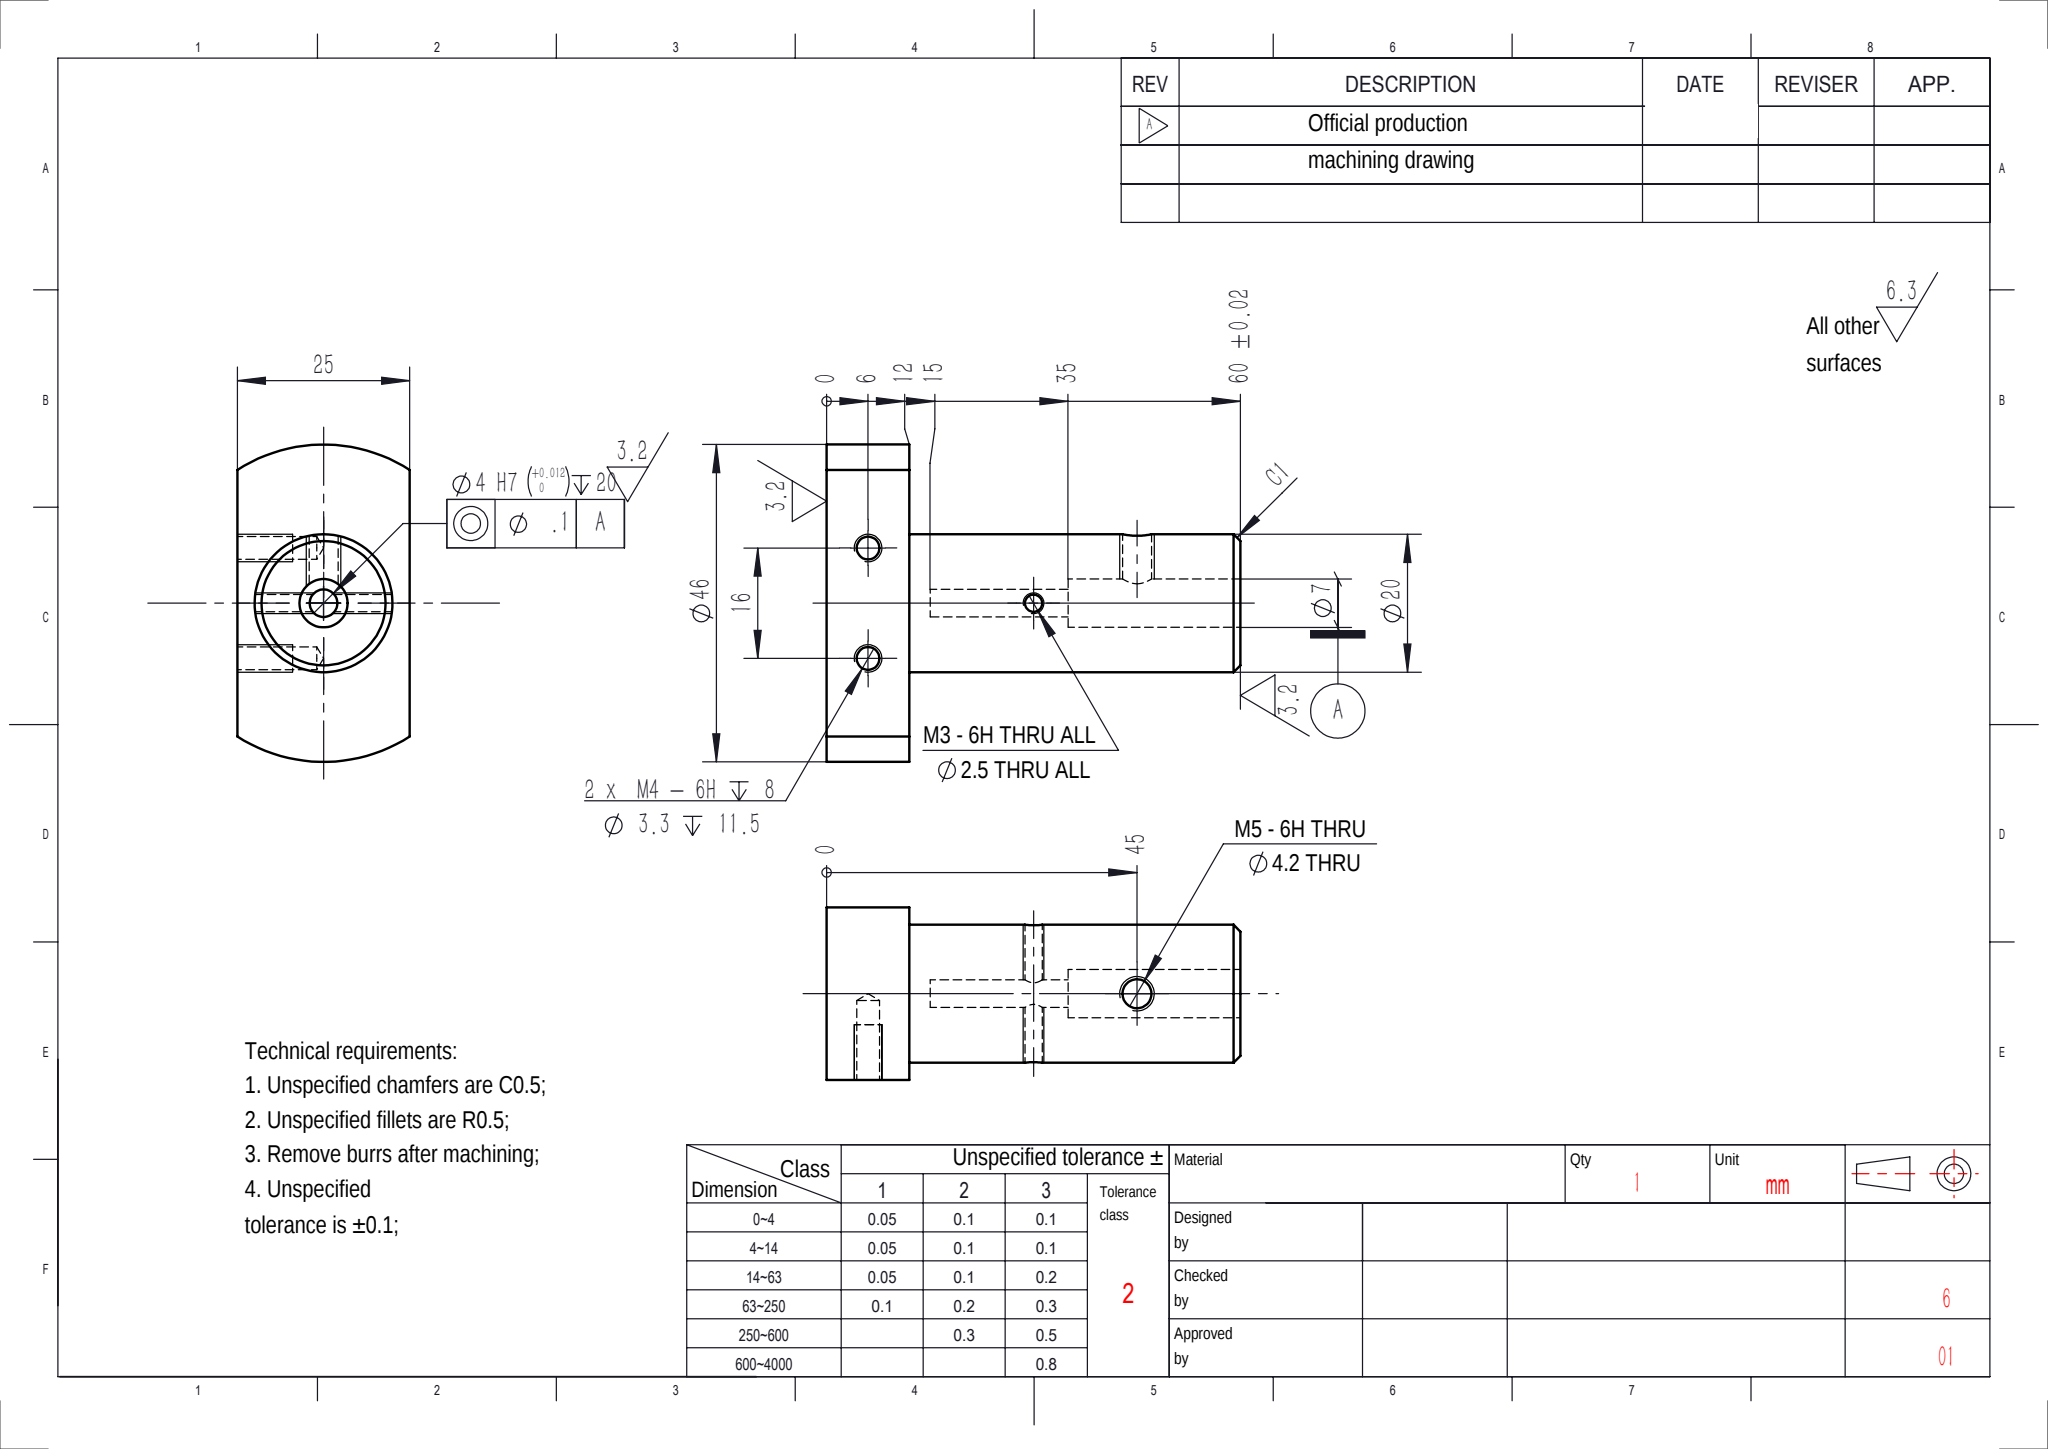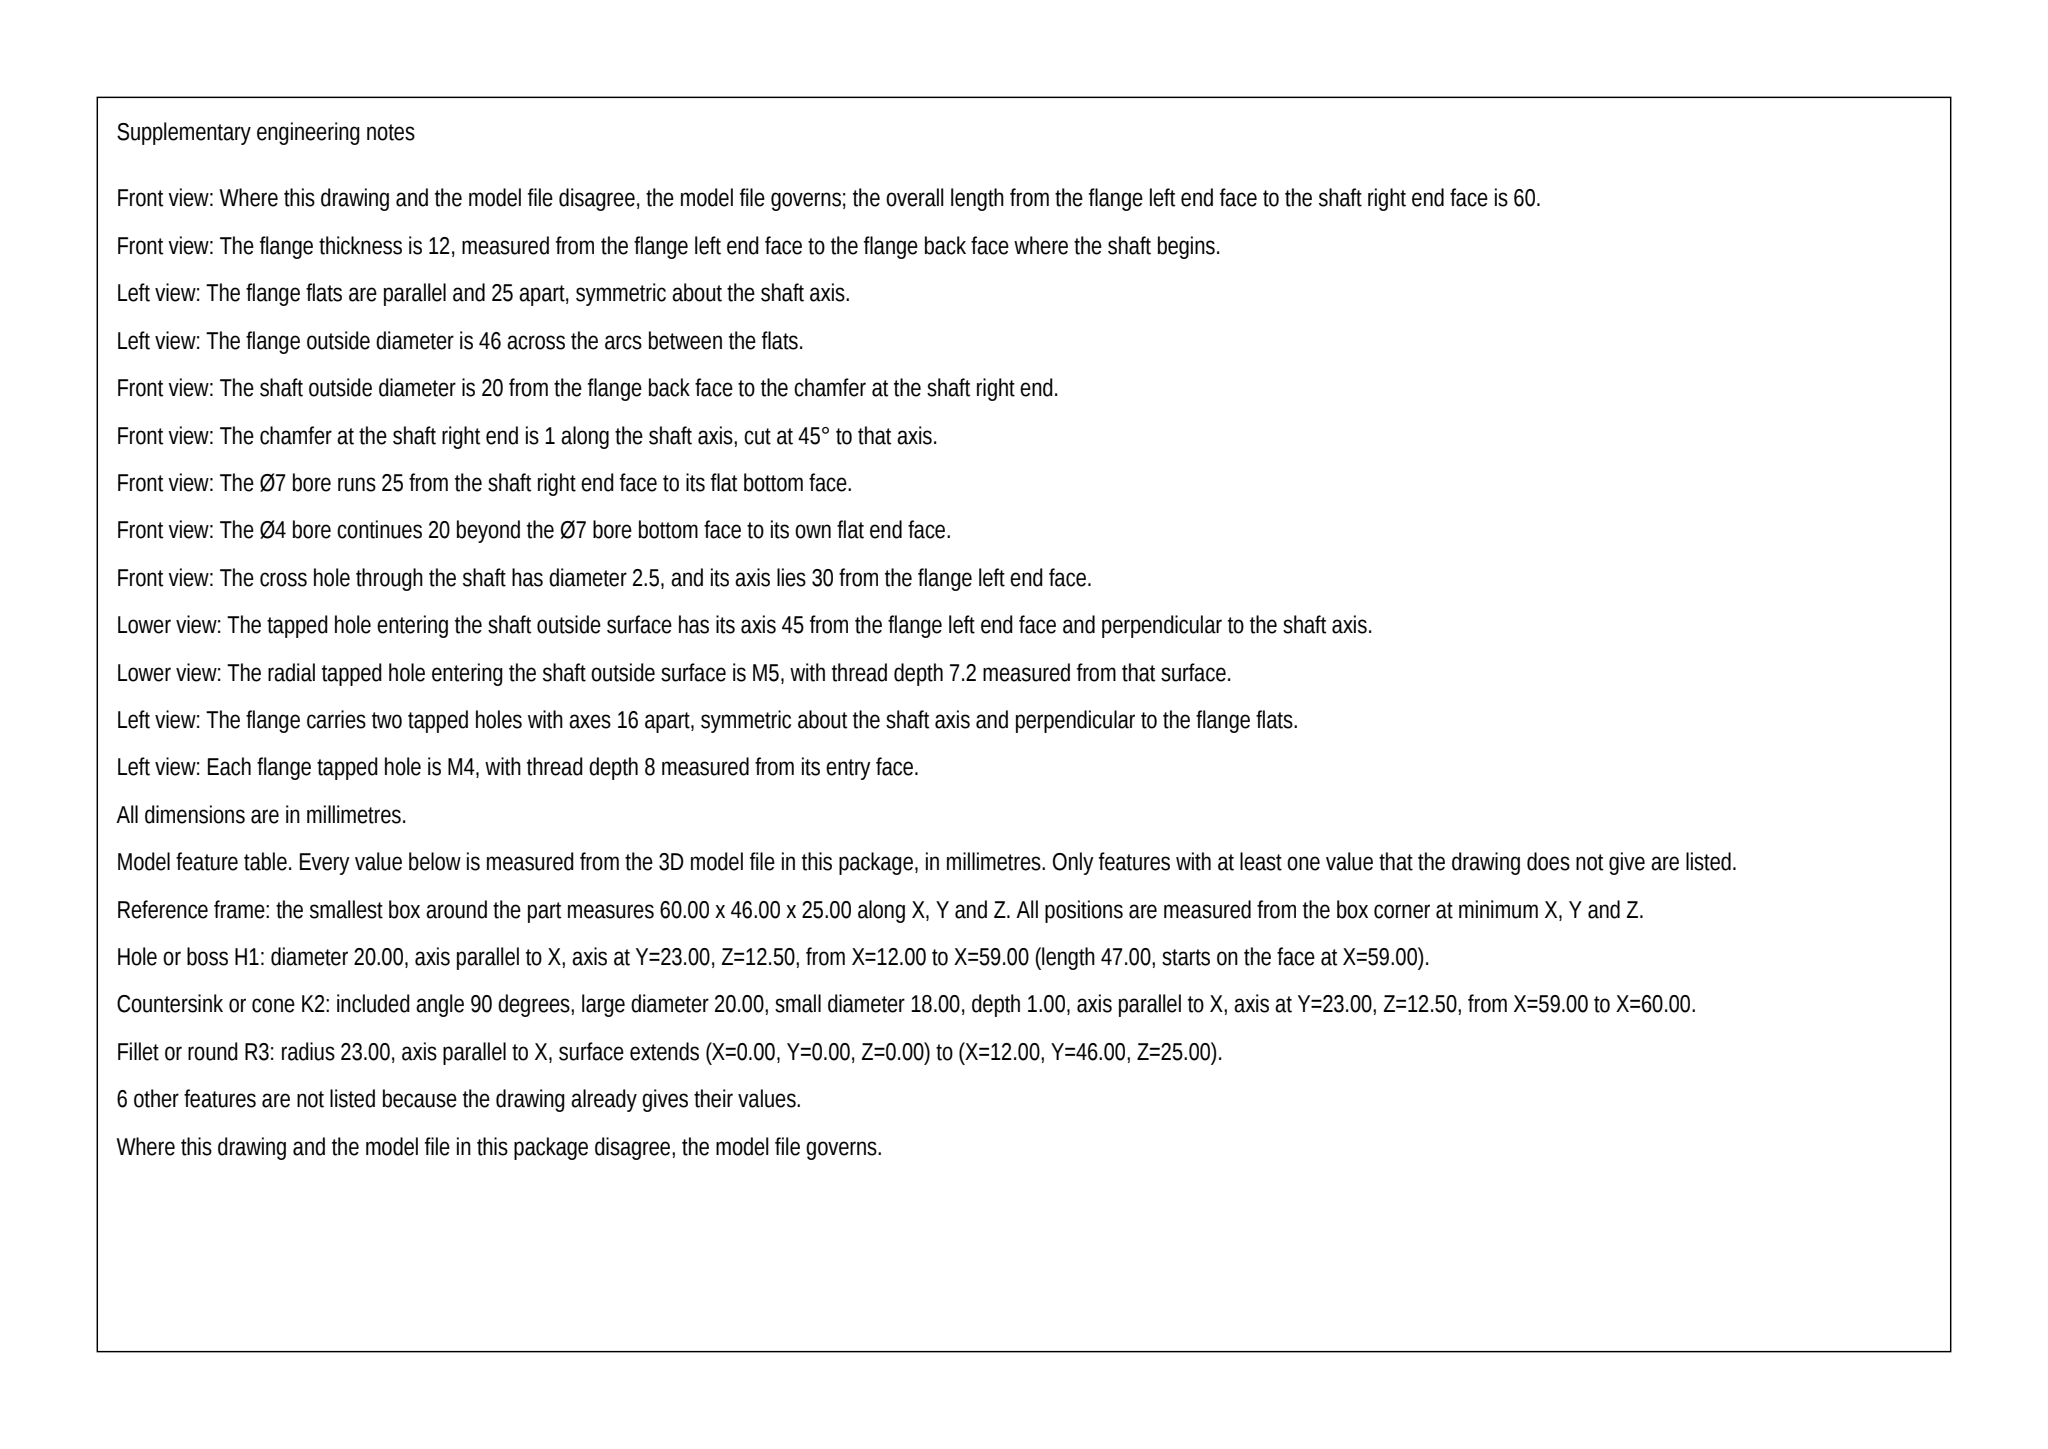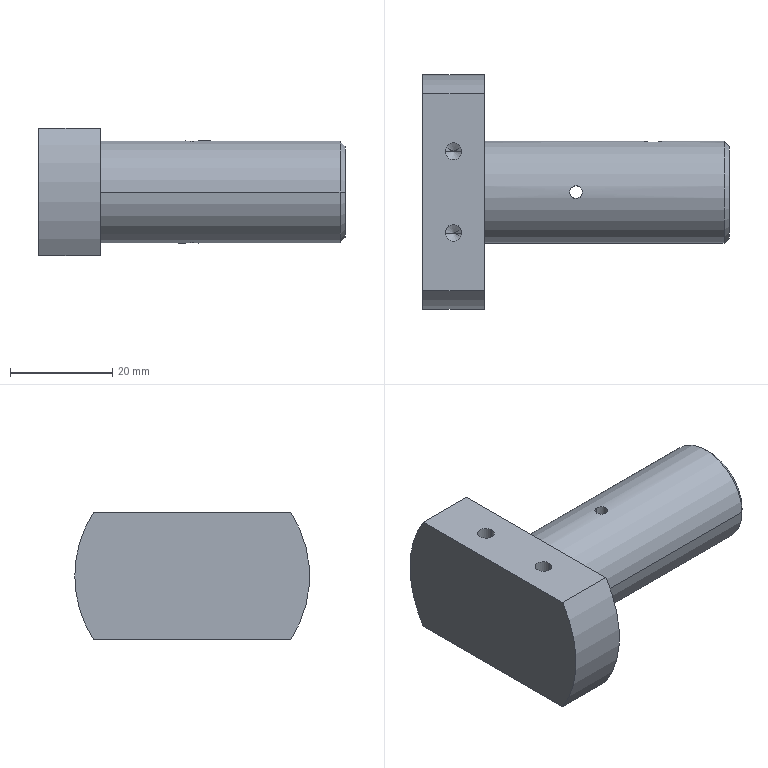Part | SolidWorks | mm | 1 solid | 32 faces | box 60 x 46 x 25 mm | volume 26549 mm3 | cylinder 19 | plane 7 | cone 6 | commonest cylinder face diameters 3.3 x4 2.5 x4 46 x3 4 x2 4.2 x2 7 x2 20 x2
build123d program:
from build123d import *

# Parameters (mm, degrees)
SKETCH2_R              = 3.5
CUT_EXTRUDE1_DEPTH     = 25
M5_TAPPED_HOLE1_REACH  = 62.357
M5_TAPPED_HOLE1_BORE_R = 2.1
SKETCH6_W              = 10.5
SKETCH6_H              = 38.613
CUT_EXTRUDE2_DEPTH     = 58.983
CHAMFER1_SIZE          = 1
SKETCH9_R              = 2
CUT_EXTRUDE3_DEPTH     = 20
M3_TAPPED_HOLE1_D      = 2.5
M4_TAPPED_HOLE1_D      = 3.3
M4_TAPPED_HOLE1_DEPTH  = 11.5
M4_TAPPED_HOLE1_TIP    = 0.9914


with BuildPart() as part:
    # Sketch1 → Revolve1 (revolve)
    with BuildSketch(Plane.XY):
        Polygon((0, 0), (0, 23), (12, 23), (12, 10), (60, 10), (60, 0), align=None)
    revolve(axis=Axis((60, 0, 0), (-1, 0, 0)))

    # Sketch2 → Cut-Extrude1 (cut)
    with BuildSketch(Plane(origin=(60, 0, 0), x_dir=(0, 0, -1), z_dir=(1, 0, 0))):
        Circle(SKETCH2_R)
    extrude(amount=-CUT_EXTRUDE1_DEPTH, mode=Mode.SUBTRACT)

    # M5 Tapped Hole1 bore (on position points) → M5 Tapped Hole1 (cut, up to next)
    with BuildSketch(Plane(origin=(45, 10, 0), x_dir=(0, 0, 1), z_dir=(0, 1, 0)), mode=Mode.PRIVATE) as m5_tapped_hole1_sk1:
        Circle(M5_TAPPED_HOLE1_BORE_R)
    m5_tapped_hole1_tool1 = extrude(m5_tapped_hole1_sk1.sketch, amount=-M5_TAPPED_HOLE1_REACH, mode=Mode.PRIVATE) & part.part
    add(m5_tapped_hole1_tool1.solids().sort_by_distance((45, 10, 0))[0], mode=Mode.SUBTRACT)

    # Sketch6 → Cut-Extrude2 (cut, through all)
    with BuildSketch(Plane(origin=(12, 0, 0), x_dir=(0, 0, -1), z_dir=(1, 0, 0))):
        with Locations((-17.75, 0)):
            Rectangle(SKETCH6_W, SKETCH6_H)
        with Locations((17.75, 0)):
            Rectangle(SKETCH6_W, SKETCH6_H)
    extrude(amount=-CUT_EXTRUDE2_DEPTH, mode=Mode.SUBTRACT)

    # Chamfer1
    chamfer1_edges = [part.edges().sort_by_distance(p)[0] for p in [
        (60, -10, 0),
    ]]
    chamfer(chamfer1_edges, length=CHAMFER1_SIZE)

    # Sketch9 → Cut-Extrude3 (cut)
    with BuildSketch(Plane(origin=(35, 0, 0), x_dir=(0, 0, -1), z_dir=(1, 0, 0))):
        Circle(SKETCH9_R)
    extrude(amount=-CUT_EXTRUDE3_DEPTH, mode=Mode.SUBTRACT)

    # M3 Tapped Hole1 (through all)
    with Locations(Plane(origin=(30, 0, -10), x_dir=(0, -1, 0), z_dir=(0, 0, -1))):
        with Locations((0, 0)):
            Hole(M3_TAPPED_HOLE1_D / 2)

    # M4 Tapped Hole1
    with Locations(Plane.XY.offset(12.5)):
        with Locations((6, -8), (6, 8)):
            Hole(M4_TAPPED_HOLE1_D / 2, depth=M4_TAPPED_HOLE1_DEPTH)
            with Locations((0, 0, -(M4_TAPPED_HOLE1_DEPTH + M4_TAPPED_HOLE1_TIP / 2))):  # 118° drill point
                Cone(0, M4_TAPPED_HOLE1_D / 2, M4_TAPPED_HOLE1_TIP, mode=Mode.SUBTRACT)


solid = part.part